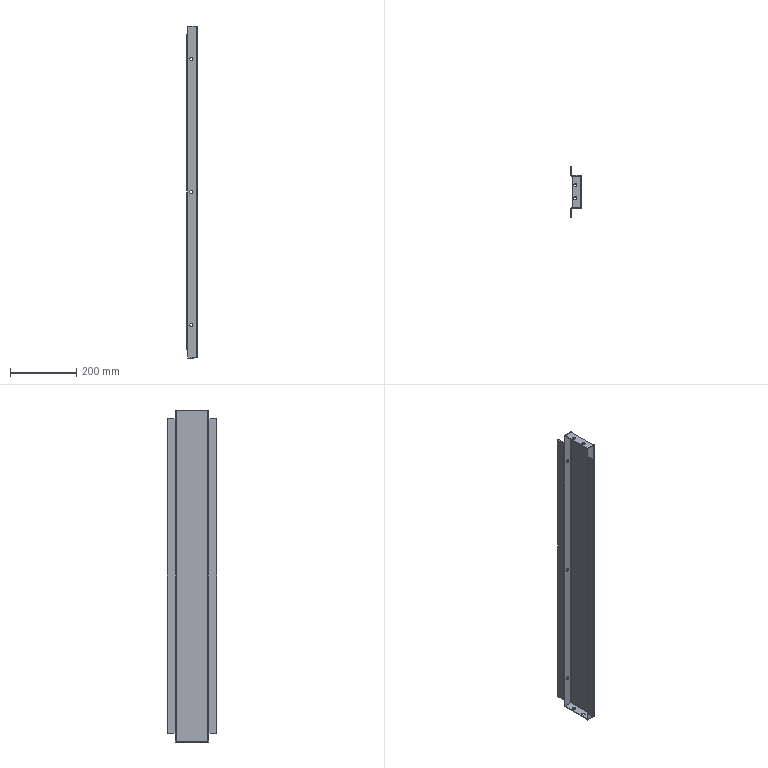Component | SolidWorks | 20LeftMiddleBeam-2 | 1 solid | 82 faces | volume 415370 mm3 | plane 50 | cylinder 32 | commonest cylinder face diameters 10 x20 6 x6 2 x6